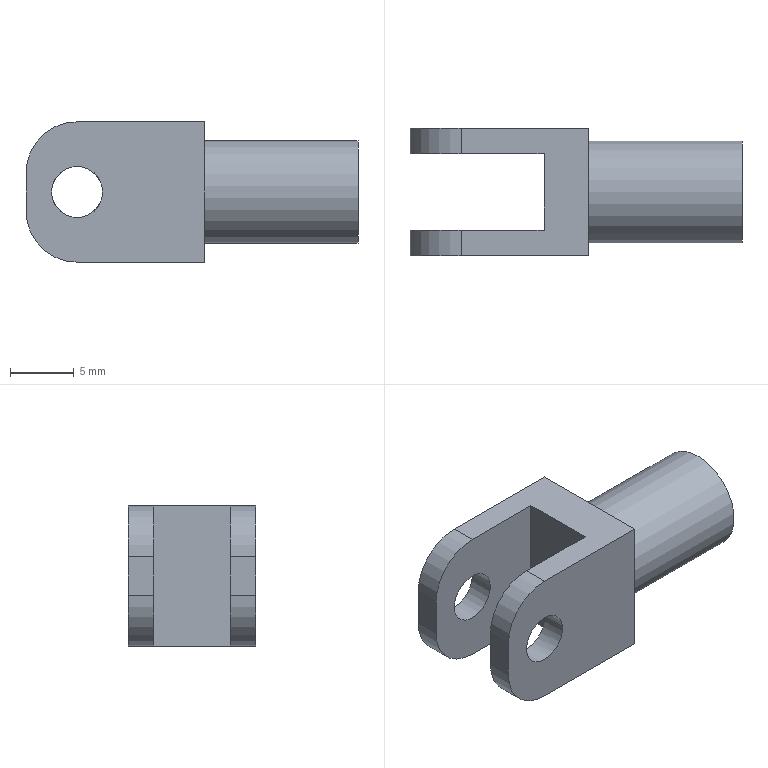Component | NX | CONNECTING_ROD_JOINT_1 | 1 solid | 20 faces | volume 1196 mm3 | plane 12 | cylinder 8 | commonest cylinder face diameters 8 x5 4 x2 5 x1